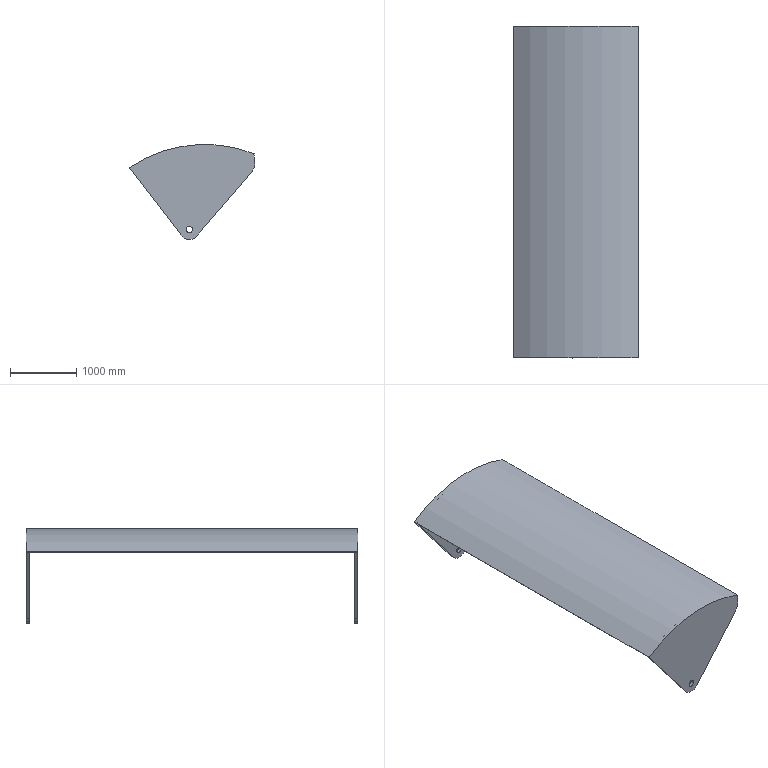Component | NX | DANGBAN | 1 solid | 24 faces | volume 316378392 mm3 | plane 14 | cylinder 10 | commonest cylinder face diameters 100 x4 400 x2 300 x2 4000 x1 4032 x1